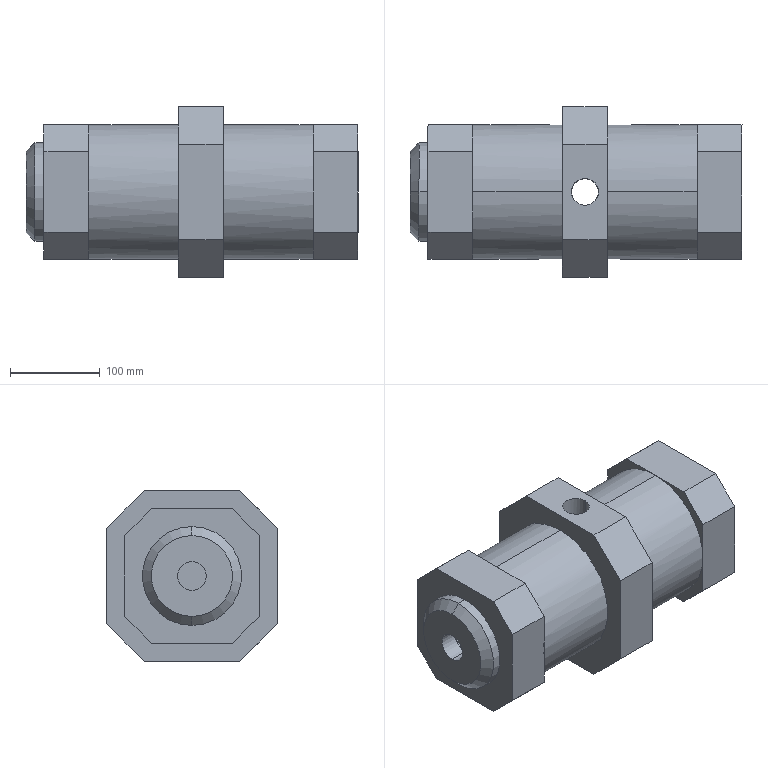Component | SolidWorks | MiddleTrunnionCylinder-1 | 1 solid | 69 faces | box 370.06 x 190.03 x 190 mm | volume 5802865 mm3 | plane 55 | cylinder 12 | cone 2 | commonest cylinder face diameters 30 x4 32 x2 110.33 x2 150 x2 80 x2 | material 45
build123d program:
from build123d import *

# Parameters (mm, degrees)
SKETCH1_W           = 150
SKETCH1_H           = 150
SKETCH1_R           = 40
BOSS_EXTRUDE1_DEPTH = 50
SKETCH2_R           = 75
SKETCH2_R_2         = 40
BOSS_EXTRUDE2_DEPTH = 250
CHAMFER1_SIZE       = 30
SKETCH3_W           = 150
SKETCH3_H           = 150
BOSS_EXTRUDE3_DEPTH = 50
CHAMFER2_SIZE       = 30
EXTRUDE_THIN1_START = 100
EXTRUDE_THIN1_DEPTH = 50
SKETCH5_R           = 15
CUT_EXTRUDE1_DEPTH  = 250
SKETCH6_R           = 55.165
SKETCH6_R_2         = 16
BOSS_EXTRUDE4_DEPTH = 20
CHAMFER3_SIZE       = 10


with BuildPart() as part:
    # Sketch1 → Boss-Extrude1 (new body)
    with BuildSketch(Plane.XY):
        with Locations((1494.26, -717)):
            Rectangle(SKETCH1_W, SKETCH1_H)
        with Locations((1494.26, -717)):
            Circle(SKETCH1_R, mode=Mode.SUBTRACT)
    extrude(amount=-BOSS_EXTRUDE1_DEPTH)

    # Sketch2 → Boss-Extrude2 (add)
    with BuildSketch(Plane(origin=(0, 0, -50), x_dir=(-1, 0, 0), z_dir=(0, 0, -1))):
        with Locations((-1494.26, -717)):
            Circle(SKETCH2_R)
        with Locations(Location((-1494.26, -717, 0), (0, 0, 180))):
            Circle(SKETCH2_R_2, mode=Mode.SUBTRACT)
    extrude(amount=BOSS_EXTRUDE2_DEPTH)

    # Chamfer1
    chamfer1_edges = [part.edges().sort_by_distance(p)[0] for p in [
        (1419.26, -642, -25),
        (1569.26, -642, -25),
        (1569.26, -792, -25),
        (1419.26, -792, -25),
    ]]
    chamfer(chamfer1_edges, length=CHAMFER1_SIZE)

    # Sketch3 → Boss-Extrude3 (add)
    with BuildSketch(Plane(origin=(0, 0, -300), x_dir=(-1, 0, 0), z_dir=(0, 0, -1))):
        with Locations((-1494.26, -717)):
            Rectangle(SKETCH3_W, SKETCH3_H)
    extrude(amount=BOSS_EXTRUDE3_DEPTH)

    # Chamfer2
    chamfer2_edges = [part.edges().sort_by_distance(p)[0] for p in [
        (1569.26, -642, -325),
        (1569.26, -792, -325),
        (1419.26, -792, -325),
        (1419.26, -642, -325),
    ]]
    chamfer(chamfer2_edges, length=CHAMFER2_SIZE)

    # Sketch4 → Extrude-Thin1 (add)
    with BuildSketch(Plane(origin=(0, 0, -50), x_dir=(-1, 0, 0), z_dir=(0, 0, -1)).offset(EXTRUDE_THIN1_START)):
        Polygon((-1547.544, -812), (-1440.975, -812), (-1399.26, -770.284), (-1399.26, -663.716), (-1440.975, -622), (-1547.544, -622), (-1589.26, -663.716), (-1589.26, -770.284), align=None)
        Polygon((-1535.117, -782), (-1453.402, -782), (-1429.26, -757.858), (-1429.26, -676.142), (-1453.402, -652), (-1535.117, -652), (-1559.26, -676.142), (-1559.26, -757.858), align=None, mode=Mode.SUBTRACT)
    extrude(amount=EXTRUDE_THIN1_DEPTH)

    # Sketch5 → Cut-Extrude1 (cut)
    with BuildSketch(Plane(origin=(1589.26, 0, 0), x_dir=(0, 0, -1), z_dir=(1, 0, 0))):
        with Locations((175, -717)):
            Circle(SKETCH5_R)
    extrude(amount=-CUT_EXTRUDE1_DEPTH, mode=Mode.SUBTRACT)

    # Sketch6 → Boss-Extrude4 (add)
    with BuildSketch(Plane.XY):
        with Locations(Location((1494.26, -717, 0), (0, 0, 180))):
            Circle(SKETCH6_R)
        with Locations((1494.26, -717)):
            Circle(SKETCH6_R_2, mode=Mode.SUBTRACT)
    extrude(amount=BOSS_EXTRUDE4_DEPTH)

    # Chamfer3
    chamfer3_edges = [part.edges().sort_by_distance(p)[0] for p in [
        (1549.425, -717, 20),
    ]]
    chamfer(chamfer3_edges, length=CHAMFER3_SIZE)


solid = part.part

# Placed as in the assembly
solid = solid.moved(Location((1715.613, -1430.899, 1234.26), (-90, -89.969, 90)))